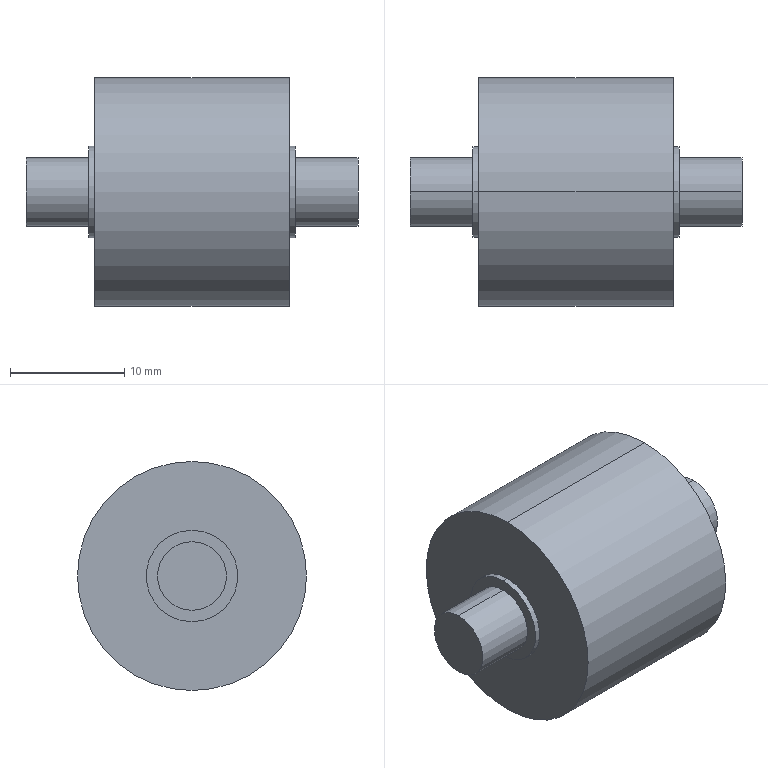Component | SolidWorks | AS-011-JG0133-1 | 1 solid | 16 faces | box 29 x 20 x 20 mm | volume 5702 mm3 | cylinder 10 | plane 6 | commonest cylinder face diameters 8 x4 6 x4 20 x2
build123d program:
from build123d import *


with BuildPart() as part:
    # Sketch1 → Revolve1 (revolve)
    with BuildSketch(Plane.XY, mode=Mode.PRIVATE) as revolve1_sk:
        Polygon((-6, 10), (-23, 10), (-23, 4), (-23.5, 4), (-23.5, 3), (-29, 3), (-29, 0), (0, 0), (0, 3), (-5.5, 3), (-5.5, 4), (-6, 4), align=None)
    revolve(revolve1_sk.sketch.rotate(Axis((-29, 0, 0), (1, 0, 0)), 90), axis=Axis((-29, 0, 0), (1, 0, 0)))


solid = part.part

# Placed as in the assembly
solid = solid.moved(Location((-0.5, -38.5, -10), (0, 0, 0)))
STEP:
#1=COLOUR_RGB('',0.7922,0.8196,0.9333);
#2=FILL_AREA_STYLE_COLOUR('',#1);
#3=FILL_AREA_STYLE('',(#2));
#4=SURFACE_STYLE_FILL_AREA(#3);
#5=SURFACE_SIDE_STYLE('',(#4));
#6=SURFACE_STYLE_USAGE(.BOTH.,#5);
#7=PRESENTATION_STYLE_ASSIGNMENT((#6));
#8=CARTESIAN_POINT('',(-0.2559,-1.516,0.));
#9=VERTEX_POINT('',#8);
#10=CARTESIAN_POINT('',(-0.2559,-1.516,-0.7874));
#11=VERTEX_POINT('',#10);
#12=CARTESIAN_POINT('',(-0.2559,-1.516,-0.3937));
#13=DIRECTION('',(-1.,0.,0.));
#14=DIRECTION('',(0.,0.,1.));
#15=AXIS2_PLACEMENT_3D('',#12,#13,#14);
#16=CIRCLE('',#15,0.3937);
#17=EDGE_CURVE('',#9,#11,#16,.T.);
#18=ORIENTED_EDGE('',*,*,#17,.T.);
#19=CARTESIAN_POINT('',(-0.9252,-1.516,-0.7874));
#20=VERTEX_POINT('',#19);
#21=CARTESIAN_POINT('',(-1.161,-1.516,-0.7874));
#22=DIRECTION('',(-1.,0.,0.));
#23=VECTOR('',#22,39.37);
#24=LINE('',#21,#23);
#25=EDGE_CURVE('',#11,#20,#24,.T.);
#26=ORIENTED_EDGE('',*,*,#25,.T.);
#27=CARTESIAN_POINT('',(-0.9252,-1.516,0.));
#28=VERTEX_POINT('',#27);
#29=CARTESIAN_POINT('',(-0.9252,-1.516,-0.3937));
#30=DIRECTION('',(-1.,0.,0.));
#31=DIRECTION('',(0.,0.,1.));
#32=AXIS2_PLACEMENT_3D('',#29,#30,#31);
#33=CIRCLE('',#32,0.3937);
#34=EDGE_CURVE('',#28,#20,#33,.T.);
#35=ORIENTED_EDGE('',*,*,#34,.F.);
#36=CARTESIAN_POINT('',(-1.161,-1.516,0.));
#37=DIRECTION('',(-1.,0.,0.));
#38=VECTOR('',#37,39.37);
#39=LINE('',#36,#38);
#40=EDGE_CURVE('',#9,#28,#39,.T.);
#41=ORIENTED_EDGE('',*,*,#40,.F.);
#42=EDGE_LOOP('',(#18,#26,#35,#41));
#43=FACE_OUTER_BOUND('',#42,.T.);
#44=CARTESIAN_POINT('',(-1.161,-1.516,-0.3937));
#45=DIRECTION('',(-1.,0.,0.));
#46=DIRECTION('',(0.,0.,1.));
#47=AXIS2_PLACEMENT_3D('',#44,#45,#46);
#48=CYLINDRICAL_SURFACE('',#47,0.3937);
#49=ADVANCED_FACE('',(#43),#48,.T.);
#50=CARTESIAN_POINT('',(-0.9252,-1.516,-0.2362));
#51=VERTEX_POINT('',#50);
#52=CARTESIAN_POINT('',(-0.9252,-1.516,-0.5512));
#53=VERTEX_POINT('',#52);
#54=CARTESIAN_POINT('',(-0.9252,-1.516,-0.3937));
#55=DIRECTION('',(-1.,0.,0.));
#56=DIRECTION('',(0.,0.,1.));
#57=AXIS2_PLACEMENT_3D('',#54,#55,#56);
#58=CIRCLE('',#57,0.1575);
#59=EDGE_CURVE('',#51,#53,#58,.T.);
#60=ORIENTED_EDGE('',*,*,#59,.T.);
#61=CARTESIAN_POINT('',(-0.9449,-1.516,-0.5512));
#62=VERTEX_POINT('',#61);
#63=CARTESIAN_POINT('',(-1.161,-1.516,-0.5512));
#64=DIRECTION('',(-1.,0.,0.));
#65=VECTOR('',#64,39.37);
#66=LINE('',#63,#65);
#67=EDGE_CURVE('',#53,#62,#66,.T.);
#68=ORIENTED_EDGE('',*,*,#67,.T.);
#69=CARTESIAN_POINT('',(-0.9449,-1.516,-0.2362));
#70=VERTEX_POINT('',#69);
#71=CARTESIAN_POINT('',(-0.9449,-1.516,-0.3937));
#72=DIRECTION('',(-1.,0.,0.));
#73=DIRECTION('',(0.,0.,1.));
#74=AXIS2_PLACEMENT_3D('',#71,#72,#73);
#75=CIRCLE('',#74,0.1575);
#76=EDGE_CURVE('',#70,#62,#75,.T.);
#77=ORIENTED_EDGE('',*,*,#76,.F.);
#78=CARTESIAN_POINT('',(-1.161,-1.516,-0.2362));
#79=DIRECTION('',(-1.,0.,0.));
#80=VECTOR('',#79,39.37);
#81=LINE('',#78,#80);
#82=EDGE_CURVE('',#51,#70,#81,.T.);
#83=ORIENTED_EDGE('',*,*,#82,.F.);
#84=EDGE_LOOP('',(#60,#68,#77,#83));
#85=FACE_OUTER_BOUND('',#84,.T.);
#86=CARTESIAN_POINT('',(-1.161,-1.516,-0.3937));
#87=DIRECTION('',(-1.,0.,0.));
#88=DIRECTION('',(0.,0.,1.));
#89=AXIS2_PLACEMENT_3D('',#86,#87,#88);
#90=CYLINDRICAL_SURFACE('',#89,0.1575);
#91=ADVANCED_FACE('',(#85),#90,.T.);
#92=CARTESIAN_POINT('',(-0.9449,-1.516,-0.2756));
#93=VERTEX_POINT('',#92);
#94=CARTESIAN_POINT('',(-0.9449,-1.516,-0.5118));
#95=VERTEX_POINT('',#94);
#96=CARTESIAN_POINT('',(-0.9449,-1.516,-0.3937));
#97=DIRECTION('',(-1.,0.,0.));
#98=DIRECTION('',(0.,0.,1.));
#99=AXIS2_PLACEMENT_3D('',#96,#97,#98);
#100=CIRCLE('',#99,0.1181);
#101=EDGE_CURVE('',#93,#95,#100,.T.);
#102=ORIENTED_EDGE('',*,*,#101,.T.);
#103=CARTESIAN_POINT('',(-1.161,-1.516,-0.5118));
#104=VERTEX_POINT('',#103);
#105=CARTESIAN_POINT('',(-1.161,-1.516,-0.5118));
#106=DIRECTION('',(-1.,0.,0.));
#107=VECTOR('',#106,39.37);
#108=LINE('',#105,#107);
#109=EDGE_CURVE('',#95,#104,#108,.T.);
#110=ORIENTED_EDGE('',*,*,#109,.T.);
#111=CARTESIAN_POINT('',(-1.161,-1.516,-0.2756));
#112=VERTEX_POINT('',#111);
#113=CARTESIAN_POINT('',(-1.161,-1.516,-0.3937));
#114=DIRECTION('',(-1.,0.,0.));
#115=DIRECTION('',(0.,0.,1.));
#116=AXIS2_PLACEMENT_3D('',#113,#114,#115);
#117=CIRCLE('',#116,0.1181);
#118=EDGE_CURVE('',#112,#104,#117,.T.);
#119=ORIENTED_EDGE('',*,*,#118,.F.);
#120=CARTESIAN_POINT('',(-1.161,-1.516,-0.2756));
#121=DIRECTION('',(-1.,0.,0.));
#122=VECTOR('',#121,39.37);
#123=LINE('',#120,#122);
#124=EDGE_CURVE('',#93,#112,#123,.T.);
#125=ORIENTED_EDGE('',*,*,#124,.F.);
#126=EDGE_LOOP('',(#102,#110,#119,#125));
#127=FACE_OUTER_BOUND('',#126,.T.);
#128=CARTESIAN_POINT('',(-1.161,-1.516,-0.3937));
#129=DIRECTION('',(-1.,0.,0.));
#130=DIRECTION('',(0.,0.,1.));
#131=AXIS2_PLACEMENT_3D('',#128,#129,#130);
#132=CYLINDRICAL_SURFACE('',#131,0.1181);
#133=ADVANCED_FACE('',(#127),#132,.T.);
#134=CARTESIAN_POINT('',(-0.01969,-1.516,-0.2756));
#135=VERTEX_POINT('',#134);
#136=CARTESIAN_POINT('',(-0.01969,-1.516,-0.5118));
#137=VERTEX_POINT('',#136);
#138=CARTESIAN_POINT('',(-0.01969,-1.516,-0.3937));
#139=DIRECTION('',(-1.,0.,0.));
#140=DIRECTION('',(0.,0.,1.));
#141=AXIS2_PLACEMENT_3D('',#138,#139,#140);
#142=CIRCLE('',#141,0.1181);
#143=EDGE_CURVE('',#135,#137,#142,.T.);
#144=ORIENTED_EDGE('',*,*,#143,.T.);
#145=CARTESIAN_POINT('',(-0.2362,-1.516,-0.5118));
#146=VERTEX_POINT('',#145);
#147=CARTESIAN_POINT('',(-1.161,-1.516,-0.5118));
#148=DIRECTION('',(-1.,0.,0.));
#149=VECTOR('',#148,39.37);
#150=LINE('',#147,#149);
#151=EDGE_CURVE('',#137,#146,#150,.T.);
#152=ORIENTED_EDGE('',*,*,#151,.T.);
#153=CARTESIAN_POINT('',(-0.2362,-1.516,-0.2756));
#154=VERTEX_POINT('',#153);
#155=CARTESIAN_POINT('',(-0.2362,-1.516,-0.3937));
#156=DIRECTION('',(-1.,0.,0.));
#157=DIRECTION('',(0.,0.,1.));
#158=AXIS2_PLACEMENT_3D('',#155,#156,#157);
#159=CIRCLE('',#158,0.1181);
#160=EDGE_CURVE('',#154,#146,#159,.T.);
#161=ORIENTED_EDGE('',*,*,#160,.F.);
#162=CARTESIAN_POINT('',(-1.161,-1.516,-0.2756));
#163=DIRECTION('',(-1.,0.,0.));
#164=VECTOR('',#163,39.37);
#165=LINE('',#162,#164);
#166=EDGE_CURVE('',#135,#154,#165,.T.);
#167=ORIENTED_EDGE('',*,*,#166,.F.);
#168=EDGE_LOOP('',(#144,#152,#161,#167));
#169=FACE_OUTER_BOUND('',#168,.T.);
#170=CARTESIAN_POINT('',(-1.161,-1.516,-0.3937));
#171=DIRECTION('',(-1.,0.,0.));
#172=DIRECTION('',(0.,0.,1.));
#173=AXIS2_PLACEMENT_3D('',#170,#171,#172);
#174=CYLINDRICAL_SURFACE('',#173,0.1181);
#175=ADVANCED_FACE('',(#169),#174,.T.);
#176=CARTESIAN_POINT('',(-0.2362,-1.516,-0.2362));
#177=VERTEX_POINT('',#176);
#178=CARTESIAN_POINT('',(-0.2362,-1.516,-0.5512));
#179=VERTEX_POINT('',#178);
#180=CARTESIAN_POINT('',(-0.2362,-1.516,-0.3937));
#181=DIRECTION('',(-1.,0.,0.));
#182=DIRECTION('',(0.,0.,1.));
#183=AXIS2_PLACEMENT_3D('',#180,#181,#182);
#184=CIRCLE('',#183,0.1575);
#185=EDGE_CURVE('',#177,#179,#184,.T.);
#186=ORIENTED_EDGE('',*,*,#185,.T.);
#187=CARTESIAN_POINT('',(-0.2559,-1.516,-0.5512));
#188=VERTEX_POINT('',#187);
#189=CARTESIAN_POINT('',(-1.161,-1.516,-0.5512));
#190=DIRECTION('',(-1.,0.,0.));
#191=VECTOR('',#190,39.37);
#192=LINE('',#189,#191);
#193=EDGE_CURVE('',#179,#188,#192,.T.);
#194=ORIENTED_EDGE('',*,*,#193,.T.);
#195=CARTESIAN_POINT('',(-0.2559,-1.516,-0.2362));
#196=VERTEX_POINT('',#195);
#197=CARTESIAN_POINT('',(-0.2559,-1.516,-0.3937));
#198=DIRECTION('',(-1.,0.,0.));
#199=DIRECTION('',(0.,0.,1.));
#200=AXIS2_PLACEMENT_3D('',#197,#198,#199);
#201=CIRCLE('',#200,0.1575);
#202=EDGE_CURVE('',#196,#188,#201,.T.);
#203=ORIENTED_EDGE('',*,*,#202,.F.);
#204=CARTESIAN_POINT('',(-1.161,-1.516,-0.2362));
#205=DIRECTION('',(-1.,0.,0.));
#206=VECTOR('',#205,39.37);
#207=LINE('',#204,#206);
#208=EDGE_CURVE('',#177,#196,#207,.T.);
#209=ORIENTED_EDGE('',*,*,#208,.F.);
#210=EDGE_LOOP('',(#186,#194,#203,#209));
#211=FACE_OUTER_BOUND('',#210,.T.);
#212=CARTESIAN_POINT('',(-1.161,-1.516,-0.3937));
#213=DIRECTION('',(-1.,0.,0.));
#214=DIRECTION('',(0.,0.,1.));
#215=AXIS2_PLACEMENT_3D('',#212,#213,#214);
#216=CYLINDRICAL_SURFACE('',#215,0.1575);
#217=ADVANCED_FACE('',(#211),#216,.T.);
#218=ORIENTED_EDGE('',*,*,#17,.F.);
#219=CARTESIAN_POINT('',(-0.2559,-1.516,-0.3937));
#220=DIRECTION('',(-1.,0.,0.));
#221=DIRECTION('',(0.,0.,1.));
#222=AXIS2_PLACEMENT_3D('',#219,#220,#221);
#223=CIRCLE('',#222,0.3937);
#224=EDGE_CURVE('',#11,#9,#223,.T.);
#225=ORIENTED_EDGE('',*,*,#224,.F.);
#226=EDGE_LOOP('',(#218,#225));
#227=FACE_OUTER_BOUND('',#226,.T.);
#228=ORIENTED_EDGE('',*,*,#202,.T.);
#229=CARTESIAN_POINT('',(-0.2559,-1.516,-0.3937));
#230=DIRECTION('',(-1.,0.,0.));
#231=DIRECTION('',(0.,0.,1.));
#232=AXIS2_PLACEMENT_3D('',#229,#230,#231);
#233=CIRCLE('',#232,0.1575);
#234=EDGE_CURVE('',#188,#196,#233,.T.);
#235=ORIENTED_EDGE('',*,*,#234,.T.);
#236=EDGE_LOOP('',(#228,#235));
#237=FACE_BOUND('',#236,.T.);
#238=CARTESIAN_POINT('',(-0.2559,-1.122,-0.3937));
#239=DIRECTION('',(-1.,0.,0.));
#240=DIRECTION('',(0.,0.,1.));
#241=AXIS2_PLACEMENT_3D('',#238,#239,#240);
#242=PLANE('',#241);
#243=ADVANCED_FACE('',(#227,#237),#242,.F.);
#244=ORIENTED_EDGE('',*,*,#193,.F.);
#245=CARTESIAN_POINT('',(-0.2362,-1.516,-0.3937));
#246=DIRECTION('',(-1.,0.,0.));
#247=DIRECTION('',(0.,0.,1.));
#248=AXIS2_PLACEMENT_3D('',#245,#246,#247);
#249=CIRCLE('',#248,0.1575);
#250=EDGE_CURVE('',#179,#177,#249,.T.);
#251=ORIENTED_EDGE('',*,*,#250,.T.);
#252=ORIENTED_EDGE('',*,*,#208,.T.);
#253=ORIENTED_EDGE('',*,*,#234,.F.);
#254=EDGE_LOOP('',(#244,#251,#252,#253));
#255=FACE_OUTER_BOUND('',#254,.T.);
#256=CARTESIAN_POINT('',(-1.161,-1.516,-0.3937));
#257=DIRECTION('',(-1.,0.,0.));
#258=DIRECTION('',(0.,0.,1.));
#259=AXIS2_PLACEMENT_3D('',#256,#257,#258);
#260=CYLINDRICAL_SURFACE('',#259,0.1575);
#261=ADVANCED_FACE('',(#255),#260,.T.);
#262=ORIENTED_EDGE('',*,*,#185,.F.);
#263=ORIENTED_EDGE('',*,*,#250,.F.);
#264=EDGE_LOOP('',(#262,#263));
#265=FACE_OUTER_BOUND('',#264,.T.);
#266=ORIENTED_EDGE('',*,*,#160,.T.);
#267=CARTESIAN_POINT('',(-0.2362,-1.516,-0.3937));
#268=DIRECTION('',(-1.,0.,0.));
#269=DIRECTION('',(0.,0.,1.));
#270=AXIS2_PLACEMENT_3D('',#267,#268,#269);
#271=CIRCLE('',#270,0.1181);
#272=EDGE_CURVE('',#146,#154,#271,.T.);
#273=ORIENTED_EDGE('',*,*,#272,.T.);
#274=EDGE_LOOP('',(#266,#273));
#275=FACE_BOUND('',#274,.T.);
#276=CARTESIAN_POINT('',(-0.2362,-1.358,-0.3937));
#277=DIRECTION('',(-1.,0.,0.));
#278=DIRECTION('',(0.,0.,1.));
#279=AXIS2_PLACEMENT_3D('',#276,#277,#278);
#280=PLANE('',#279);
#281=ADVANCED_FACE('',(#265,#275),#280,.F.);
#282=ORIENTED_EDGE('',*,*,#151,.F.);
#283=CARTESIAN_POINT('',(-0.01969,-1.516,-0.3937));
#284=DIRECTION('',(-1.,0.,0.));
#285=DIRECTION('',(0.,0.,1.));
#286=AXIS2_PLACEMENT_3D('',#283,#284,#285);
#287=CIRCLE('',#286,0.1181);
#288=EDGE_CURVE('',#137,#135,#287,.T.);
#289=ORIENTED_EDGE('',*,*,#288,.T.);
#290=ORIENTED_EDGE('',*,*,#166,.T.);
#291=ORIENTED_EDGE('',*,*,#272,.F.);
#292=EDGE_LOOP('',(#282,#289,#290,#291));
#293=FACE_OUTER_BOUND('',#292,.T.);
#294=CARTESIAN_POINT('',(-1.161,-1.516,-0.3937));
#295=DIRECTION('',(-1.,0.,0.));
#296=DIRECTION('',(0.,0.,1.));
#297=AXIS2_PLACEMENT_3D('',#294,#295,#296);
#298=CYLINDRICAL_SURFACE('',#297,0.1181);
#299=ADVANCED_FACE('',(#293),#298,.T.);
#300=ORIENTED_EDGE('',*,*,#143,.F.);
#301=ORIENTED_EDGE('',*,*,#288,.F.);
#302=EDGE_LOOP('',(#300,#301));
#303=FACE_OUTER_BOUND('',#302,.T.);
#304=CARTESIAN_POINT('',(-0.01969,-1.398,-0.3937));
#305=DIRECTION('',(-1.,0.,0.));
#306=DIRECTION('',(0.,0.,1.));
#307=AXIS2_PLACEMENT_3D('',#304,#305,#306);
#308=PLANE('',#307);
#309=ADVANCED_FACE('',(#303),#308,.F.);
#310=ORIENTED_EDGE('',*,*,#118,.T.);
#311=CARTESIAN_POINT('',(-1.161,-1.516,-0.3937));
#312=DIRECTION('',(-1.,0.,0.));
#313=DIRECTION('',(0.,0.,1.));
#314=AXIS2_PLACEMENT_3D('',#311,#312,#313);
#315=CIRCLE('',#314,0.1181);
#316=EDGE_CURVE('',#104,#112,#315,.T.);
#317=ORIENTED_EDGE('',*,*,#316,.T.);
#318=EDGE_LOOP('',(#310,#317));
#319=FACE_OUTER_BOUND('',#318,.T.);
#320=CARTESIAN_POINT('',(-1.161,-1.398,-0.3937));
#321=DIRECTION('',(1.,0.,0.));
#322=DIRECTION('',(0.,0.,-1.));
#323=AXIS2_PLACEMENT_3D('',#320,#321,#322);
#324=PLANE('',#323);
#325=ADVANCED_FACE('',(#319),#324,.F.);
#326=ORIENTED_EDGE('',*,*,#109,.F.);
#327=CARTESIAN_POINT('',(-0.9449,-1.516,-0.3937));
#328=DIRECTION('',(-1.,0.,0.));
#329=DIRECTION('',(0.,0.,1.));
#330=AXIS2_PLACEMENT_3D('',#327,#328,#329);
#331=CIRCLE('',#330,0.1181);
#332=EDGE_CURVE('',#95,#93,#331,.T.);
#333=ORIENTED_EDGE('',*,*,#332,.T.);
#334=ORIENTED_EDGE('',*,*,#124,.T.);
#335=ORIENTED_EDGE('',*,*,#316,.F.);
#336=EDGE_LOOP('',(#326,#333,#334,#335));
#337=FACE_OUTER_BOUND('',#336,.T.);
#338=CARTESIAN_POINT('',(-1.161,-1.516,-0.3937));
#339=DIRECTION('',(-1.,0.,0.));
#340=DIRECTION('',(0.,0.,1.));
#341=AXIS2_PLACEMENT_3D('',#338,#339,#340);
#342=CYLINDRICAL_SURFACE('',#341,0.1181);
#343=ADVANCED_FACE('',(#337),#342,.T.);
#344=ORIENTED_EDGE('',*,*,#101,.F.);
#345=ORIENTED_EDGE('',*,*,#332,.F.);
#346=EDGE_LOOP('',(#344,#345));
#347=FACE_BOUND('',#346,.T.);
#348=ORIENTED_EDGE('',*,*,#76,.T.);
#349=CARTESIAN_POINT('',(-0.9449,-1.516,-0.3937));
#350=DIRECTION('',(-1.,0.,0.));
#351=DIRECTION('',(0.,0.,1.));
#352=AXIS2_PLACEMENT_3D('',#349,#350,#351);
#353=CIRCLE('',#352,0.1575);
#354=EDGE_CURVE('',#62,#70,#353,.T.);
#355=ORIENTED_EDGE('',*,*,#354,.T.);
#356=EDGE_LOOP('',(#348,#355));
#357=FACE_OUTER_BOUND('',#356,.T.);
#358=CARTESIAN_POINT('',(-0.9449,-1.358,-0.3937));
#359=DIRECTION('',(1.,0.,0.));
#360=DIRECTION('',(0.,0.,-1.));
#361=AXIS2_PLACEMENT_3D('',#358,#359,#360);
#362=PLANE('',#361);
#363=ADVANCED_FACE('',(#347,#357),#362,.F.);
#364=ORIENTED_EDGE('',*,*,#67,.F.);
#365=CARTESIAN_POINT('',(-0.9252,-1.516,-0.3937));
#366=DIRECTION('',(-1.,0.,0.));
#367=DIRECTION('',(0.,0.,1.));
#368=AXIS2_PLACEMENT_3D('',#365,#366,#367);
#369=CIRCLE('',#368,0.1575);
#370=EDGE_CURVE('',#53,#51,#369,.T.);
#371=ORIENTED_EDGE('',*,*,#370,.T.);
#372=ORIENTED_EDGE('',*,*,#82,.T.);
#373=ORIENTED_EDGE('',*,*,#354,.F.);
#374=EDGE_LOOP('',(#364,#371,#372,#373));
#375=FACE_OUTER_BOUND('',#374,.T.);
#376=CARTESIAN_POINT('',(-1.161,-1.516,-0.3937));
#377=DIRECTION('',(-1.,0.,0.));
#378=DIRECTION('',(0.,0.,1.));
#379=AXIS2_PLACEMENT_3D('',#376,#377,#378);
#380=CYLINDRICAL_SURFACE('',#379,0.1575);
#381=ADVANCED_FACE('',(#375),#380,.T.);
#382=ORIENTED_EDGE('',*,*,#59,.F.);
#383=ORIENTED_EDGE('',*,*,#370,.F.);
#384=EDGE_LOOP('',(#382,#383));
#385=FACE_BOUND('',#384,.T.);
#386=ORIENTED_EDGE('',*,*,#34,.T.);
#387=CARTESIAN_POINT('',(-0.9252,-1.516,-0.3937));
#388=DIRECTION('',(-1.,0.,0.));
#389=DIRECTION('',(0.,0.,1.));
#390=AXIS2_PLACEMENT_3D('',#387,#388,#389);
#391=CIRCLE('',#390,0.3937);
#392=EDGE_CURVE('',#20,#28,#391,.T.);
#393=ORIENTED_EDGE('',*,*,#392,.T.);
#394=EDGE_LOOP('',(#386,#393));
#395=FACE_OUTER_BOUND('',#394,.T.);
#396=CARTESIAN_POINT('',(-0.9252,-1.122,-0.3937));
#397=DIRECTION('',(1.,0.,0.));
#398=DIRECTION('',(0.,0.,-1.));
#399=AXIS2_PLACEMENT_3D('',#396,#397,#398);
#400=PLANE('',#399);
#401=ADVANCED_FACE('',(#385,#395),#400,.F.);
#402=ORIENTED_EDGE('',*,*,#25,.F.);
#403=ORIENTED_EDGE('',*,*,#224,.T.);
#404=ORIENTED_EDGE('',*,*,#40,.T.);
#405=ORIENTED_EDGE('',*,*,#392,.F.);
#406=EDGE_LOOP('',(#402,#403,#404,#405));
#407=FACE_OUTER_BOUND('',#406,.T.);
#408=CARTESIAN_POINT('',(-1.161,-1.516,-0.3937));
#409=DIRECTION('',(-1.,0.,0.));
#410=DIRECTION('',(0.,0.,1.));
#411=AXIS2_PLACEMENT_3D('',#408,#409,#410);
#412=CYLINDRICAL_SURFACE('',#411,0.3937);
#413=ADVANCED_FACE('',(#407),#412,.T.);
#414=CLOSED_SHELL('',(#49,#91,#133,#175,#217,#243,#261,#281,#299,#309,#325,#343,#363,#381,#401,#413));
#415=MANIFOLD_SOLID_BREP('',#414);
#416=STYLED_ITEM('',(#7),#415);
#417=PRESENTATION_LAYER_ASSIGNMENT('','',(#416));
#418=CARTESIAN_POINT('',(0.,0.,0.));
#419=DIRECTION('',(0.,0.,1.));
#420=DIRECTION('',(1.,0.,0.));
#421=AXIS2_PLACEMENT_3D('',#418,#419,#420);
#422=(LENGTH_UNIT()NAMED_UNIT(*)SI_UNIT($,.METRE.));
#423=LENGTH_MEASURE_WITH_UNIT(LENGTH_MEASURE(0.0254),#422);
#424=DIMENSIONAL_EXPONENTS(1.,0.,0.,0.,0.,0.,0.);
#425=(CONVERSION_BASED_UNIT('',#423)LENGTH_UNIT()NAMED_UNIT(#424));
#426=UNCERTAINTY_MEASURE_WITH_UNIT(LENGTH_MEASURE(0.00001),#425,'','');
#427=(NAMED_UNIT(*)PLANE_ANGLE_UNIT()SI_UNIT($,.RADIAN.));
#428=(NAMED_UNIT(*)SI_UNIT($,.STERADIAN.)SOLID_ANGLE_UNIT());
#429=(GEOMETRIC_REPRESENTATION_CONTEXT(3)GLOBAL_UNCERTAINTY_ASSIGNED_CONTEXT((#426))GLOBAL_UNIT_ASSIGNED_CONTEXT((#425,#427,#428))REPRESENTATION_CONTEXT('',''));
#430=ADVANCED_BREP_SHAPE_REPRESENTATION('',(#415,#421),#429);
#431=(LENGTH_UNIT()NAMED_UNIT(*)SI_UNIT($,.METRE.));
#432=LENGTH_MEASURE_WITH_UNIT(LENGTH_MEASURE(0.0254),#431);
#433=DIMENSIONAL_EXPONENTS(1.,0.,0.,0.,0.,0.,0.);
#434=(CONVERSION_BASED_UNIT('',#432)LENGTH_UNIT()NAMED_UNIT(#433));
#435=UNCERTAINTY_MEASURE_WITH_UNIT(LENGTH_MEASURE(0.00001),#434,'','');
#436=(NAMED_UNIT(*)PLANE_ANGLE_UNIT()SI_UNIT($,.RADIAN.));
#437=(NAMED_UNIT(*)SI_UNIT($,.STERADIAN.)SOLID_ANGLE_UNIT());
#438=(GEOMETRIC_REPRESENTATION_CONTEXT(3)GLOBAL_UNCERTAINTY_ASSIGNED_CONTEXT((#435))GLOBAL_UNIT_ASSIGNED_CONTEXT((#434,#436,#437))REPRESENTATION_CONTEXT('',''));
#439=MECHANICAL_DESIGN_GEOMETRIC_PRESENTATION_REPRESENTATION('',(#416),#438);